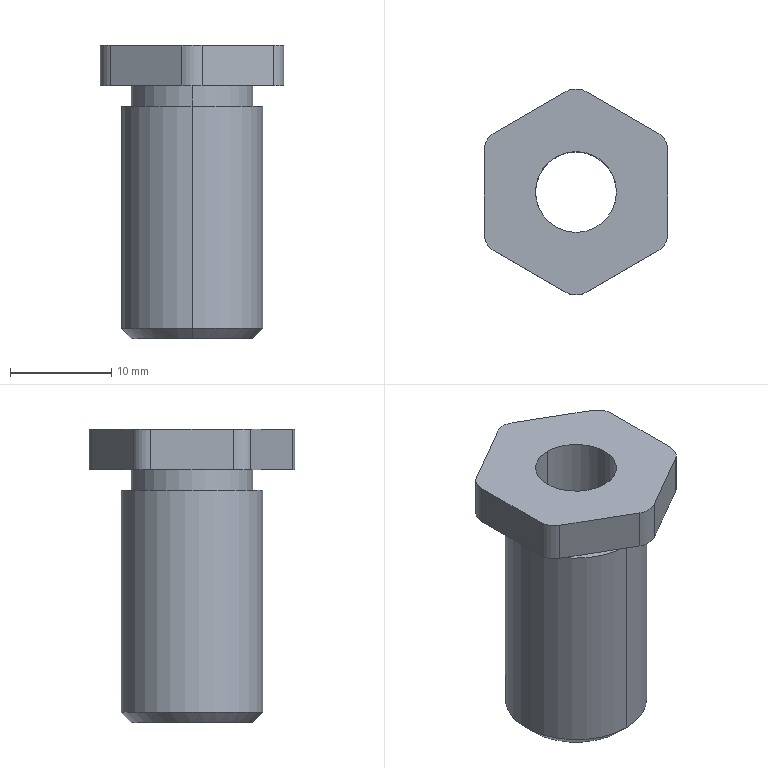CAM job | Mastercam | mm | 3 operations | part box 18.19 x 20.38 x 29
1. 2D High Speed (2D Dynamic Mill) | 6 - 6 平铣刀
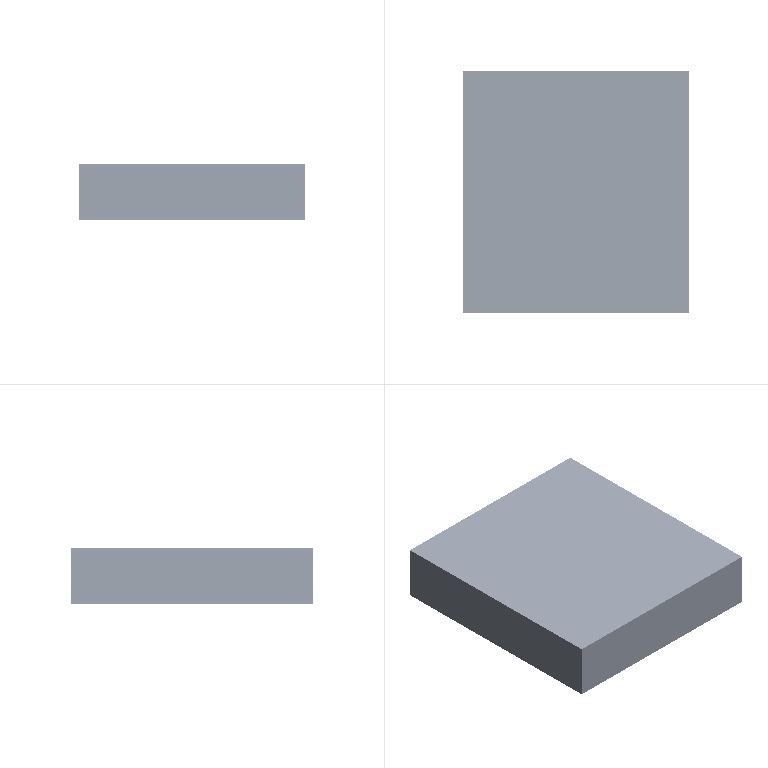2. Contour (2D) | 6 - 6 平铣刀
3. Contour (2D chamfer) | 7 - 4 倒角刀